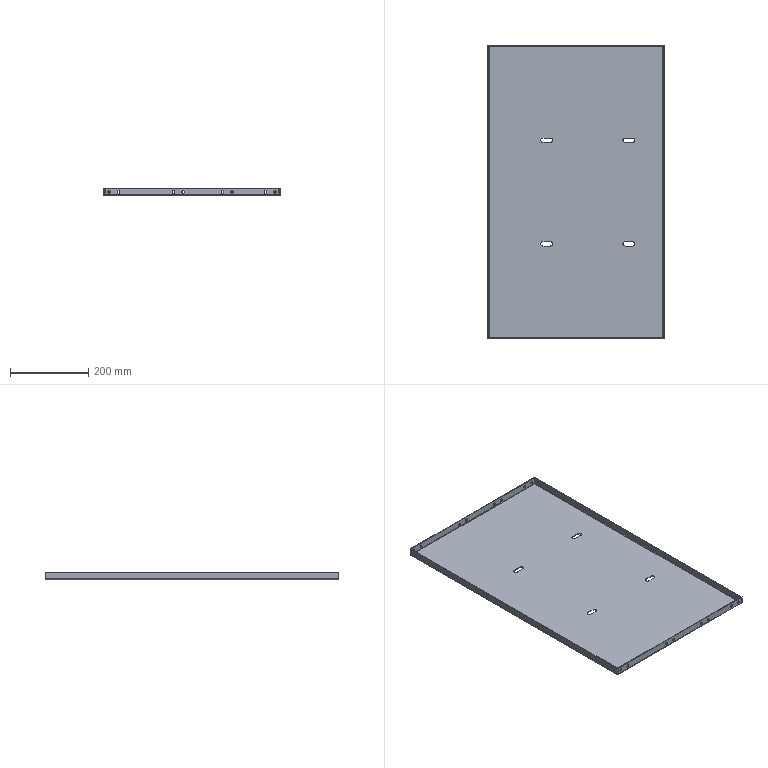Component | SolidWorks | Partition(No.29)-1 | 1 solid | 90 faces | volume 753374 mm3 | cylinder 48 | plane 42 | commonest cylinder face diameters 6.5 x32 11 x8 6 x4 2 x4 | material Plain Carbon Steel